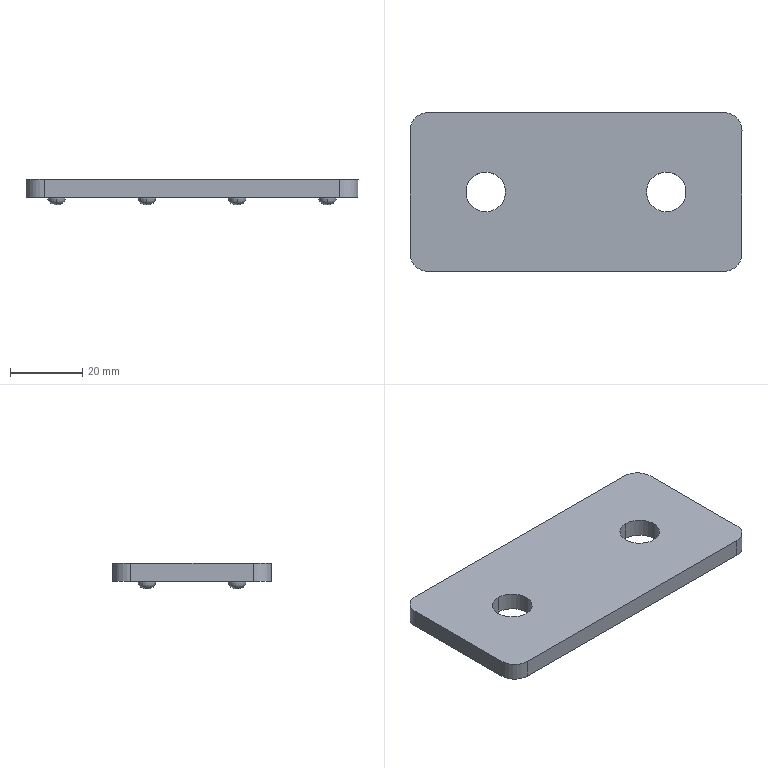Component | SolidWorks | G-Beam-1_BeamEndPlate-1 | 1 solid | 38 faces | box 92 x 44 x 7 mm | volume 19408 mm3 | torus 16 | plane 14 | cylinder 8 | commonest cylinder face diameters 11 x4 10 x4 | material Plain Carbon Steel
STEP:
#1=COLOUR_RGB('',0.7922,0.8196,0.9333);
#2=FILL_AREA_STYLE_COLOUR('',#1);
#3=FILL_AREA_STYLE('',(#2));
#4=SURFACE_STYLE_FILL_AREA(#3);
#5=SURFACE_SIDE_STYLE('',(#4));
#6=SURFACE_STYLE_USAGE(.BOTH.,#5);
#7=PRESENTATION_STYLE_ASSIGNMENT((#6));
#8=CARTESIAN_POINT('',(-170.63,344.077,264.226));
#9=VERTEX_POINT('',#8);
#10=CARTESIAN_POINT('',(-170.63,344.274,264.226));
#11=VERTEX_POINT('',#10);
#12=CARTESIAN_POINT('',(-170.63,344.176,264.226));
#13=DIRECTION('',(-0.,0.,-1.));
#14=DIRECTION('',(-0.,-1.,0.));
#15=AXIS2_PLACEMENT_3D('',#12,#13,#14);
#16=CIRCLE('',#15,0.09843);
#17=EDGE_CURVE('',#9,#11,#16,.T.);
#18=ORIENTED_EDGE('',*,*,#17,.T.);
#19=CARTESIAN_POINT('',(-170.63,344.195,264.147));
#20=VERTEX_POINT('',#19);
#21=CARTESIAN_POINT('',(-170.63,344.195,264.226));
#22=DIRECTION('',(-1.,0.,0.));
#23=DIRECTION('',(0.,0.,1.));
#24=AXIS2_PLACEMENT_3D('',#21,#22,#23);
#25=CIRCLE('',#24,0.07874);
#26=EDGE_CURVE('',#11,#20,#25,.T.);
#27=ORIENTED_EDGE('',*,*,#26,.T.);
#28=CARTESIAN_POINT('',(-170.63,344.156,264.147));
#29=VERTEX_POINT('',#28);
#30=CARTESIAN_POINT('',(-170.63,344.176,264.147));
#31=DIRECTION('',(-0.,0.,-1.));
#32=DIRECTION('',(-0.,-1.,0.));
#33=AXIS2_PLACEMENT_3D('',#30,#31,#32);
#34=CIRCLE('',#33,0.01969);
#35=EDGE_CURVE('',#29,#20,#34,.T.);
#36=ORIENTED_EDGE('',*,*,#35,.F.);
#37=CARTESIAN_POINT('',(-170.63,344.156,264.226));
#38=DIRECTION('',(1.,-0.,-0.));
#39=DIRECTION('',(-0.,0.,-1.));
#40=AXIS2_PLACEMENT_3D('',#37,#38,#39);
#41=CIRCLE('',#40,0.07874);
#42=EDGE_CURVE('',#9,#29,#41,.T.);
#43=ORIENTED_EDGE('',*,*,#42,.F.);
#44=EDGE_LOOP('',(#18,#27,#36,#43));
#45=FACE_OUTER_BOUND('',#44,.T.);
#46=CARTESIAN_POINT('',(-170.63,344.176,264.226));
#47=DIRECTION('',(-0.,0.,-1.));
#48=DIRECTION('',(-0.,-1.,-0.));
#49=AXIS2_PLACEMENT_3D('',#46,#47,#48);
#50=TOROIDAL_SURFACE('',#49,0.01969,0.07874);
#51=ADVANCED_FACE('',(#45),#50,.T.);
#52=CARTESIAN_POINT('',(-170.63,345.062,264.226));
#53=VERTEX_POINT('',#52);
#54=CARTESIAN_POINT('',(-170.63,345.258,264.226));
#55=VERTEX_POINT('',#54);
#56=CARTESIAN_POINT('',(-170.63,345.16,264.226));
#57=DIRECTION('',(-0.,0.,-1.));
#58=DIRECTION('',(-0.,-1.,0.));
#59=AXIS2_PLACEMENT_3D('',#56,#57,#58);
#60=CIRCLE('',#59,0.09843);
#61=EDGE_CURVE('',#53,#55,#60,.T.);
#62=ORIENTED_EDGE('',*,*,#61,.T.);
#63=CARTESIAN_POINT('',(-170.63,345.18,264.147));
#64=VERTEX_POINT('',#63);
#65=CARTESIAN_POINT('',(-170.63,345.18,264.226));
#66=DIRECTION('',(-1.,0.,0.));
#67=DIRECTION('',(0.,0.,1.));
#68=AXIS2_PLACEMENT_3D('',#65,#66,#67);
#69=CIRCLE('',#68,0.07874);
#70=EDGE_CURVE('',#55,#64,#69,.T.);
#71=ORIENTED_EDGE('',*,*,#70,.T.);
#72=CARTESIAN_POINT('',(-170.63,345.14,264.147));
#73=VERTEX_POINT('',#72);
#74=CARTESIAN_POINT('',(-170.63,345.16,264.147));
#75=DIRECTION('',(-0.,0.,-1.));
#76=DIRECTION('',(-0.,-1.,0.));
#77=AXIS2_PLACEMENT_3D('',#74,#75,#76);
#78=CIRCLE('',#77,0.01969);
#79=EDGE_CURVE('',#73,#64,#78,.T.);
#80=ORIENTED_EDGE('',*,*,#79,.F.);
#81=CARTESIAN_POINT('',(-170.63,345.14,264.226));
#82=DIRECTION('',(1.,-0.,-0.));
#83=DIRECTION('',(-0.,0.,-1.));
#84=AXIS2_PLACEMENT_3D('',#81,#82,#83);
#85=CIRCLE('',#84,0.07874);
#86=EDGE_CURVE('',#53,#73,#85,.T.);
#87=ORIENTED_EDGE('',*,*,#86,.F.);
#88=EDGE_LOOP('',(#62,#71,#80,#87));
#89=FACE_OUTER_BOUND('',#88,.T.);
#90=CARTESIAN_POINT('',(-170.63,345.16,264.226));
#91=DIRECTION('',(-0.,0.,-1.));
#92=DIRECTION('',(-0.,-1.,-0.));
#93=AXIS2_PLACEMENT_3D('',#90,#91,#92);
#94=TOROIDAL_SURFACE('',#93,0.01969,0.07874);
#95=ADVANCED_FACE('',(#89),#94,.T.);
#96=CARTESIAN_POINT('',(-171.614,344.077,264.226));
#97=VERTEX_POINT('',#96);
#98=CARTESIAN_POINT('',(-171.614,344.274,264.226));
#99=VERTEX_POINT('',#98);
#100=CARTESIAN_POINT('',(-171.614,344.176,264.226));
#101=DIRECTION('',(-0.,0.,-1.));
#102=DIRECTION('',(-0.,-1.,0.));
#103=AXIS2_PLACEMENT_3D('',#100,#101,#102);
#104=CIRCLE('',#103,0.09843);
#105=EDGE_CURVE('',#97,#99,#104,.T.);
#106=ORIENTED_EDGE('',*,*,#105,.T.);
#107=CARTESIAN_POINT('',(-171.614,344.195,264.147));
#108=VERTEX_POINT('',#107);
#109=CARTESIAN_POINT('',(-171.614,344.195,264.226));
#110=DIRECTION('',(-1.,0.,0.));
#111=DIRECTION('',(0.,0.,1.));
#112=AXIS2_PLACEMENT_3D('',#109,#110,#111);
#113=CIRCLE('',#112,0.07874);
#114=EDGE_CURVE('',#99,#108,#113,.T.);
#115=ORIENTED_EDGE('',*,*,#114,.T.);
#116=CARTESIAN_POINT('',(-171.614,344.156,264.147));
#117=VERTEX_POINT('',#116);
#118=CARTESIAN_POINT('',(-171.614,344.176,264.147));
#119=DIRECTION('',(-0.,0.,-1.));
#120=DIRECTION('',(-0.,-1.,0.));
#121=AXIS2_PLACEMENT_3D('',#118,#119,#120);
#122=CIRCLE('',#121,0.01969);
#123=EDGE_CURVE('',#117,#108,#122,.T.);
#124=ORIENTED_EDGE('',*,*,#123,.F.);
#125=CARTESIAN_POINT('',(-171.614,344.156,264.226));
#126=DIRECTION('',(1.,-0.,-0.));
#127=DIRECTION('',(-0.,0.,-1.));
#128=AXIS2_PLACEMENT_3D('',#125,#126,#127);
#129=CIRCLE('',#128,0.07874);
#130=EDGE_CURVE('',#97,#117,#129,.T.);
#131=ORIENTED_EDGE('',*,*,#130,.F.);
#132=EDGE_LOOP('',(#106,#115,#124,#131));
#133=FACE_OUTER_BOUND('',#132,.T.);
#134=CARTESIAN_POINT('',(-171.614,344.176,264.226));
#135=DIRECTION('',(-0.,0.,-1.));
#136=DIRECTION('',(-0.,-1.,-0.));
#137=AXIS2_PLACEMENT_3D('',#134,#135,#136);
#138=TOROIDAL_SURFACE('',#137,0.01969,0.07874);
#139=ADVANCED_FACE('',(#133),#138,.T.);
#140=CARTESIAN_POINT('',(-171.614,345.062,264.226));
#141=VERTEX_POINT('',#140);
#142=CARTESIAN_POINT('',(-171.614,345.258,264.226));
#143=VERTEX_POINT('',#142);
#144=CARTESIAN_POINT('',(-171.614,345.16,264.226));
#145=DIRECTION('',(-0.,0.,-1.));
#146=DIRECTION('',(-0.,-1.,0.));
#147=AXIS2_PLACEMENT_3D('',#144,#145,#146);
#148=CIRCLE('',#147,0.09843);
#149=EDGE_CURVE('',#141,#143,#148,.T.);
#150=ORIENTED_EDGE('',*,*,#149,.T.);
#151=CARTESIAN_POINT('',(-171.614,345.18,264.147));
#152=VERTEX_POINT('',#151);
#153=CARTESIAN_POINT('',(-171.614,345.18,264.226));
#154=DIRECTION('',(-1.,0.,0.));
#155=DIRECTION('',(0.,0.,1.));
#156=AXIS2_PLACEMENT_3D('',#153,#154,#155);
#157=CIRCLE('',#156,0.07874);
#158=EDGE_CURVE('',#143,#152,#157,.T.);
#159=ORIENTED_EDGE('',*,*,#158,.T.);
#160=CARTESIAN_POINT('',(-171.614,345.14,264.147));
#161=VERTEX_POINT('',#160);
#162=CARTESIAN_POINT('',(-171.614,345.16,264.147));
#163=DIRECTION('',(-0.,0.,-1.));
#164=DIRECTION('',(-0.,-1.,0.));
#165=AXIS2_PLACEMENT_3D('',#162,#163,#164);
#166=CIRCLE('',#165,0.01969);
#167=EDGE_CURVE('',#161,#152,#166,.T.);
#168=ORIENTED_EDGE('',*,*,#167,.F.);
#169=CARTESIAN_POINT('',(-171.614,345.14,264.226));
#170=DIRECTION('',(1.,-0.,-0.));
#171=DIRECTION('',(-0.,0.,-1.));
#172=AXIS2_PLACEMENT_3D('',#169,#170,#171);
#173=CIRCLE('',#172,0.07874);
#174=EDGE_CURVE('',#141,#161,#173,.T.);
#175=ORIENTED_EDGE('',*,*,#174,.F.);
#176=EDGE_LOOP('',(#150,#159,#168,#175));
#177=FACE_OUTER_BOUND('',#176,.T.);
#178=CARTESIAN_POINT('',(-171.614,345.16,264.226));
#179=DIRECTION('',(-0.,0.,-1.));
#180=DIRECTION('',(-0.,-1.,-0.));
#181=AXIS2_PLACEMENT_3D('',#178,#179,#180);
#182=TOROIDAL_SURFACE('',#181,0.01969,0.07874);
#183=ADVANCED_FACE('',(#177),#182,.T.);
#184=CARTESIAN_POINT('',(-172.599,344.156,264.147));
#185=VERTEX_POINT('',#184);
#186=CARTESIAN_POINT('',(-172.599,344.195,264.147));
#187=VERTEX_POINT('',#186);
#188=CARTESIAN_POINT('',(-172.599,344.176,264.147));
#189=DIRECTION('',(-0.,0.,-1.));
#190=DIRECTION('',(0.,1.,0.));
#191=AXIS2_PLACEMENT_3D('',#188,#189,#190);
#192=CIRCLE('',#191,0.01969);
#193=EDGE_CURVE('',#185,#187,#192,.T.);
#194=ORIENTED_EDGE('',*,*,#193,.F.);
#195=CARTESIAN_POINT('',(-172.599,344.077,264.226));
#196=VERTEX_POINT('',#195);
#197=CARTESIAN_POINT('',(-172.599,344.156,264.226));
#198=DIRECTION('',(-1.,0.,0.));
#199=DIRECTION('',(0.,0.,1.));
#200=AXIS2_PLACEMENT_3D('',#197,#198,#199);
#201=CIRCLE('',#200,0.07874);
#202=EDGE_CURVE('',#185,#196,#201,.T.);
#203=ORIENTED_EDGE('',*,*,#202,.T.);
#204=CARTESIAN_POINT('',(-172.599,344.274,264.226));
#205=VERTEX_POINT('',#204);
#206=CARTESIAN_POINT('',(-172.599,344.176,264.226));
#207=DIRECTION('',(-0.,0.,-1.));
#208=DIRECTION('',(-0.,-1.,0.));
#209=AXIS2_PLACEMENT_3D('',#206,#207,#208);
#210=CIRCLE('',#209,0.09843);
#211=EDGE_CURVE('',#196,#205,#210,.T.);
#212=ORIENTED_EDGE('',*,*,#211,.T.);
#213=CARTESIAN_POINT('',(-172.599,344.195,264.226));
#214=DIRECTION('',(1.,-0.,-0.));
#215=DIRECTION('',(-0.,0.,-1.));
#216=AXIS2_PLACEMENT_3D('',#213,#214,#215);
#217=CIRCLE('',#216,0.07874);
#218=EDGE_CURVE('',#187,#205,#217,.T.);
#219=ORIENTED_EDGE('',*,*,#218,.F.);
#220=EDGE_LOOP('',(#194,#203,#212,#219));
#221=FACE_OUTER_BOUND('',#220,.T.);
#222=CARTESIAN_POINT('',(-172.599,344.176,264.226));
#223=DIRECTION('',(0.,-0.,1.));
#224=DIRECTION('',(0.,1.,0.));
#225=AXIS2_PLACEMENT_3D('',#222,#223,#224);
#226=TOROIDAL_SURFACE('',#225,0.01969,0.07874);
#227=ADVANCED_FACE('',(#221),#226,.T.);
#228=CARTESIAN_POINT('',(-172.599,345.14,264.147));
#229=VERTEX_POINT('',#228);
#230=CARTESIAN_POINT('',(-172.599,345.18,264.147));
#231=VERTEX_POINT('',#230);
#232=CARTESIAN_POINT('',(-172.599,345.16,264.147));
#233=DIRECTION('',(-0.,0.,-1.));
#234=DIRECTION('',(0.,1.,0.));
#235=AXIS2_PLACEMENT_3D('',#232,#233,#234);
#236=CIRCLE('',#235,0.01969);
#237=EDGE_CURVE('',#229,#231,#236,.T.);
#238=ORIENTED_EDGE('',*,*,#237,.F.);
#239=CARTESIAN_POINT('',(-172.599,345.062,264.226));
#240=VERTEX_POINT('',#239);
#241=CARTESIAN_POINT('',(-172.599,345.14,264.226));
#242=DIRECTION('',(-1.,0.,0.));
#243=DIRECTION('',(0.,0.,1.));
#244=AXIS2_PLACEMENT_3D('',#241,#242,#243);
#245=CIRCLE('',#244,0.07874);
#246=EDGE_CURVE('',#229,#240,#245,.T.);
#247=ORIENTED_EDGE('',*,*,#246,.T.);
#248=CARTESIAN_POINT('',(-172.599,345.258,264.226));
#249=VERTEX_POINT('',#248);
#250=CARTESIAN_POINT('',(-172.599,345.16,264.226));
#251=DIRECTION('',(-0.,0.,-1.));
#252=DIRECTION('',(-0.,-1.,0.));
#253=AXIS2_PLACEMENT_3D('',#250,#251,#252);
#254=CIRCLE('',#253,0.09843);
#255=EDGE_CURVE('',#240,#249,#254,.T.);
#256=ORIENTED_EDGE('',*,*,#255,.T.);
#257=CARTESIAN_POINT('',(-172.599,345.18,264.226));
#258=DIRECTION('',(1.,-0.,-0.));
#259=DIRECTION('',(-0.,0.,-1.));
#260=AXIS2_PLACEMENT_3D('',#257,#258,#259);
#261=CIRCLE('',#260,0.07874);
#262=EDGE_CURVE('',#231,#249,#261,.T.);
#263=ORIENTED_EDGE('',*,*,#262,.F.);
#264=EDGE_LOOP('',(#238,#247,#256,#263));
#265=FACE_OUTER_BOUND('',#264,.T.);
#266=CARTESIAN_POINT('',(-172.599,345.16,264.226));
#267=DIRECTION('',(0.,-0.,1.));
#268=DIRECTION('',(0.,1.,0.));
#269=AXIS2_PLACEMENT_3D('',#266,#267,#268);
#270=TOROIDAL_SURFACE('',#269,0.01969,0.07874);
#271=ADVANCED_FACE('',(#265),#270,.T.);
#272=CARTESIAN_POINT('',(-173.583,344.156,264.147));
#273=VERTEX_POINT('',#272);
#274=CARTESIAN_POINT('',(-173.583,344.195,264.147));
#275=VERTEX_POINT('',#274);
#276=CARTESIAN_POINT('',(-173.583,344.176,264.147));
#277=DIRECTION('',(-0.,0.,-1.));
#278=DIRECTION('',(0.,1.,0.));
#279=AXIS2_PLACEMENT_3D('',#276,#277,#278);
#280=CIRCLE('',#279,0.01969);
#281=EDGE_CURVE('',#273,#275,#280,.T.);
#282=ORIENTED_EDGE('',*,*,#281,.F.);
#283=CARTESIAN_POINT('',(-173.583,344.077,264.226));
#284=VERTEX_POINT('',#283);
#285=CARTESIAN_POINT('',(-173.583,344.156,264.226));
#286=DIRECTION('',(-1.,0.,0.));
#287=DIRECTION('',(0.,0.,1.));
#288=AXIS2_PLACEMENT_3D('',#285,#286,#287);
#289=CIRCLE('',#288,0.07874);
#290=EDGE_CURVE('',#273,#284,#289,.T.);
#291=ORIENTED_EDGE('',*,*,#290,.T.);
#292=CARTESIAN_POINT('',(-173.583,344.274,264.226));
#293=VERTEX_POINT('',#292);
#294=CARTESIAN_POINT('',(-173.583,344.176,264.226));
#295=DIRECTION('',(-0.,0.,-1.));
#296=DIRECTION('',(-0.,-1.,0.));
#297=AXIS2_PLACEMENT_3D('',#294,#295,#296);
#298=CIRCLE('',#297,0.09843);
#299=EDGE_CURVE('',#284,#293,#298,.T.);
#300=ORIENTED_EDGE('',*,*,#299,.T.);
#301=CARTESIAN_POINT('',(-173.583,344.195,264.226));
#302=DIRECTION('',(1.,-0.,-0.));
#303=DIRECTION('',(-0.,0.,-1.));
#304=AXIS2_PLACEMENT_3D('',#301,#302,#303);
#305=CIRCLE('',#304,0.07874);
#306=EDGE_CURVE('',#275,#293,#305,.T.);
#307=ORIENTED_EDGE('',*,*,#306,.F.);
#308=EDGE_LOOP('',(#282,#291,#300,#307));
#309=FACE_OUTER_BOUND('',#308,.T.);
#310=CARTESIAN_POINT('',(-173.583,344.176,264.226));
#311=DIRECTION('',(0.,-0.,1.));
#312=DIRECTION('',(0.,1.,0.));
#313=AXIS2_PLACEMENT_3D('',#310,#311,#312);
#314=TOROIDAL_SURFACE('',#313,0.01969,0.07874);
#315=ADVANCED_FACE('',(#309),#314,.T.);
#316=CARTESIAN_POINT('',(-173.583,345.14,264.147));
#317=VERTEX_POINT('',#316);
#318=CARTESIAN_POINT('',(-173.583,345.18,264.147));
#319=VERTEX_POINT('',#318);
#320=CARTESIAN_POINT('',(-173.583,345.16,264.147));
#321=DIRECTION('',(-0.,0.,-1.));
#322=DIRECTION('',(0.,1.,0.));
#323=AXIS2_PLACEMENT_3D('',#320,#321,#322);
#324=CIRCLE('',#323,0.01969);
#325=EDGE_CURVE('',#317,#319,#324,.T.);
#326=ORIENTED_EDGE('',*,*,#325,.F.);
#327=CARTESIAN_POINT('',(-173.583,345.062,264.226));
#328=VERTEX_POINT('',#327);
#329=CARTESIAN_POINT('',(-173.583,345.14,264.226));
#330=DIRECTION('',(-1.,0.,0.));
#331=DIRECTION('',(0.,0.,1.));
#332=AXIS2_PLACEMENT_3D('',#329,#330,#331);
#333=CIRCLE('',#332,0.07874);
#334=EDGE_CURVE('',#317,#328,#333,.T.);
#335=ORIENTED_EDGE('',*,*,#334,.T.);
#336=CARTESIAN_POINT('',(-173.583,345.258,264.226));
#337=VERTEX_POINT('',#336);
#338=CARTESIAN_POINT('',(-173.583,345.16,264.226));
#339=DIRECTION('',(-0.,0.,-1.));
#340=DIRECTION('',(-0.,-1.,0.));
#341=AXIS2_PLACEMENT_3D('',#338,#339,#340);
#342=CIRCLE('',#341,0.09843);
#343=EDGE_CURVE('',#328,#337,#342,.T.);
#344=ORIENTED_EDGE('',*,*,#343,.T.);
#345=CARTESIAN_POINT('',(-173.583,345.18,264.226));
#346=DIRECTION('',(1.,-0.,-0.));
#347=DIRECTION('',(-0.,0.,-1.));
#348=AXIS2_PLACEMENT_3D('',#345,#346,#347);
#349=CIRCLE('',#348,0.07874);
#350=EDGE_CURVE('',#319,#337,#349,.T.);
#351=ORIENTED_EDGE('',*,*,#350,.F.);
#352=EDGE_LOOP('',(#326,#335,#344,#351));
#353=FACE_OUTER_BOUND('',#352,.T.);
#354=CARTESIAN_POINT('',(-173.583,345.16,264.226));
#355=DIRECTION('',(0.,-0.,1.));
#356=DIRECTION('',(0.,1.,0.));
#357=AXIS2_PLACEMENT_3D('',#354,#355,#356);
#358=TOROIDAL_SURFACE('',#357,0.01969,0.07874);
#359=ADVANCED_FACE('',(#353),#358,.T.);
#360=CARTESIAN_POINT('',(-173.091,344.884,264.226));
#361=VERTEX_POINT('',#360);
#362=CARTESIAN_POINT('',(-173.091,344.451,264.226));
#363=VERTEX_POINT('',#362);
#364=CARTESIAN_POINT('',(-173.091,344.668,264.226));
#365=DIRECTION('',(-0.,0.,-1.));
#366=DIRECTION('',(-0.,-1.,0.));
#367=AXIS2_PLACEMENT_3D('',#364,#365,#366);
#368=CIRCLE('',#367,0.2165);
#369=EDGE_CURVE('',#361,#363,#368,.T.);
#370=ORIENTED_EDGE('',*,*,#369,.T.);
#371=CARTESIAN_POINT('',(-173.091,344.451,264.423));
#372=VERTEX_POINT('',#371);
#373=CARTESIAN_POINT('',(-173.091,344.451,264.226));
#374=DIRECTION('',(0.,-0.,1.));
#375=VECTOR('',#374,39.37);
#376=LINE('',#373,#375);
#377=EDGE_CURVE('',#363,#372,#376,.T.);
#378=ORIENTED_EDGE('',*,*,#377,.T.);
#379=CARTESIAN_POINT('',(-173.091,344.884,264.423));
#380=VERTEX_POINT('',#379);
#381=CARTESIAN_POINT('',(-173.091,344.668,264.423));
#382=DIRECTION('',(-0.,0.,-1.));
#383=DIRECTION('',(-0.,-1.,0.));
#384=AXIS2_PLACEMENT_3D('',#381,#382,#383);
#385=CIRCLE('',#384,0.2165);
#386=EDGE_CURVE('',#380,#372,#385,.T.);
#387=ORIENTED_EDGE('',*,*,#386,.F.);
#388=CARTESIAN_POINT('',(-173.091,344.884,264.226));
#389=DIRECTION('',(0.,-0.,1.));
#390=VECTOR('',#389,39.37);
#391=LINE('',#388,#390);
#392=EDGE_CURVE('',#361,#380,#391,.T.);
#393=ORIENTED_EDGE('',*,*,#392,.F.);
#394=EDGE_LOOP('',(#370,#378,#387,#393));
#395=FACE_OUTER_BOUND('',#394,.T.);
#396=CARTESIAN_POINT('',(-173.091,344.668,264.226));
#397=DIRECTION('',(0.,-0.,1.));
#398=DIRECTION('',(0.,1.,0.));
#399=AXIS2_PLACEMENT_3D('',#396,#397,#398);
#400=CYLINDRICAL_SURFACE('',#399,0.2165);
#401=ADVANCED_FACE('',(#395),#400,.F.);
#402=CARTESIAN_POINT('',(-171.122,344.884,264.226));
#403=VERTEX_POINT('',#402);
#404=CARTESIAN_POINT('',(-171.122,344.451,264.226));
#405=VERTEX_POINT('',#404);
#406=CARTESIAN_POINT('',(-171.122,344.668,264.226));
#407=DIRECTION('',(-0.,0.,-1.));
#408=DIRECTION('',(-0.,-1.,0.));
#409=AXIS2_PLACEMENT_3D('',#406,#407,#408);
#410=CIRCLE('',#409,0.2165);
#411=EDGE_CURVE('',#403,#405,#410,.T.);
#412=ORIENTED_EDGE('',*,*,#411,.T.);
#413=CARTESIAN_POINT('',(-171.122,344.451,264.423));
#414=VERTEX_POINT('',#413);
#415=CARTESIAN_POINT('',(-171.122,344.451,264.226));
#416=DIRECTION('',(0.,-0.,1.));
#417=VECTOR('',#416,39.37);
#418=LINE('',#415,#417);
#419=EDGE_CURVE('',#405,#414,#418,.T.);
#420=ORIENTED_EDGE('',*,*,#419,.T.);
#421=CARTESIAN_POINT('',(-171.122,344.884,264.423));
#422=VERTEX_POINT('',#421);
#423=CARTESIAN_POINT('',(-171.122,344.668,264.423));
#424=DIRECTION('',(-0.,0.,-1.));
#425=DIRECTION('',(-0.,-1.,0.));
#426=AXIS2_PLACEMENT_3D('',#423,#424,#425);
#427=CIRCLE('',#426,0.2165);
#428=EDGE_CURVE('',#422,#414,#427,.T.);
#429=ORIENTED_EDGE('',*,*,#428,.F.);
#430=CARTESIAN_POINT('',(-171.122,344.884,264.226));
#431=DIRECTION('',(0.,-0.,1.));
#432=VECTOR('',#431,39.37);
#433=LINE('',#430,#432);
#434=EDGE_CURVE('',#403,#422,#433,.T.);
#435=ORIENTED_EDGE('',*,*,#434,.F.);
#436=EDGE_LOOP('',(#412,#420,#429,#435));
#437=FACE_OUTER_BOUND('',#436,.T.);
#438=CARTESIAN_POINT('',(-171.122,344.668,264.226));
#439=DIRECTION('',(0.,-0.,1.));
#440=DIRECTION('',(0.,1.,0.));
#441=AXIS2_PLACEMENT_3D('',#438,#439,#440);
#442=CYLINDRICAL_SURFACE('',#441,0.2165);
#443=ADVANCED_FACE('',(#437),#442,.F.);
#444=CARTESIAN_POINT('',(-172.599,345.16,264.226));
#445=DIRECTION('',(-0.,0.,-1.));
#446=DIRECTION('',(-0.,-1.,0.));
#447=AXIS2_PLACEMENT_3D('',#444,#445,#446);
#448=CIRCLE('',#447,0.09843);
#449=EDGE_CURVE('',#249,#240,#448,.T.);
#450=ORIENTED_EDGE('',*,*,#449,.F.);
#451=ORIENTED_EDGE('',*,*,#255,.F.);
#452=EDGE_LOOP('',(#450,#451));
#453=FACE_BOUND('',#452,.T.);
#454=ORIENTED_EDGE('',*,*,#17,.F.);
#455=CARTESIAN_POINT('',(-170.63,344.176,264.226));
#456=DIRECTION('',(-0.,0.,-1.));
#457=DIRECTION('',(-0.,-1.,0.));
#458=AXIS2_PLACEMENT_3D('',#455,#456,#457);
#459=CIRCLE('',#458,0.09843);
#460=EDGE_CURVE('',#11,#9,#459,.T.);
#461=ORIENTED_EDGE('',*,*,#460,.F.);
#462=EDGE_LOOP('',(#454,#461));
#463=FACE_BOUND('',#462,.T.);
#464=ORIENTED_EDGE('',*,*,#61,.F.);
#465=CARTESIAN_POINT('',(-170.63,345.16,264.226));
#466=DIRECTION('',(-0.,0.,-1.));
#467=DIRECTION('',(-0.,-1.,0.));
#468=AXIS2_PLACEMENT_3D('',#465,#466,#467);
#469=CIRCLE('',#468,0.09843);
#470=EDGE_CURVE('',#55,#53,#469,.T.);
#471=ORIENTED_EDGE('',*,*,#470,.F.);
#472=EDGE_LOOP('',(#464,#471));
#473=FACE_BOUND('',#472,.T.);
#474=ORIENTED_EDGE('',*,*,#105,.F.);
#475=CARTESIAN_POINT('',(-171.614,344.176,264.226));
#476=DIRECTION('',(-0.,0.,-1.));
#477=DIRECTION('',(-0.,-1.,0.));
#478=AXIS2_PLACEMENT_3D('',#475,#476,#477);
#479=CIRCLE('',#478,0.09843);
#480=EDGE_CURVE('',#99,#97,#479,.T.);
#481=ORIENTED_EDGE('',*,*,#480,.F.);
#482=EDGE_LOOP('',(#474,#481));
#483=FACE_BOUND('',#482,.T.);
#484=CARTESIAN_POINT('',(-172.599,344.176,264.226));
#485=DIRECTION('',(-0.,0.,-1.));
#486=DIRECTION('',(-0.,-1.,0.));
#487=AXIS2_PLACEMENT_3D('',#484,#485,#486);
#488=CIRCLE('',#487,0.09843);
#489=EDGE_CURVE('',#205,#196,#488,.T.);
#490=ORIENTED_EDGE('',*,*,#489,.F.);
#491=ORIENTED_EDGE('',*,*,#211,.F.);
#492=EDGE_LOOP('',(#490,#491));
#493=FACE_BOUND('',#492,.T.);
#494=CARTESIAN_POINT('',(-173.583,344.176,264.226));
#495=DIRECTION('',(-0.,0.,-1.));
#496=DIRECTION('',(-0.,-1.,0.));
#497=AXIS2_PLACEMENT_3D('',#494,#495,#496);
#498=CIRCLE('',#497,0.09843);
#499=EDGE_CURVE('',#293,#284,#498,.T.);
#500=ORIENTED_EDGE('',*,*,#499,.F.);
#501=ORIENTED_EDGE('',*,*,#299,.F.);
#502=EDGE_LOOP('',(#500,#501));
#503=FACE_BOUND('',#502,.T.);
#504=CARTESIAN_POINT('',(-173.583,345.16,264.226));
#505=DIRECTION('',(-0.,0.,-1.));
#506=DIRECTION('',(-0.,-1.,0.));
#507=AXIS2_PLACEMENT_3D('',#504,#505,#506);
#508=CIRCLE('',#507,0.09843);
#509=EDGE_CURVE('',#337,#328,#508,.T.);
#510=ORIENTED_EDGE('',*,*,#509,.F.);
#511=ORIENTED_EDGE('',*,*,#343,.F.);
#512=EDGE_LOOP('',(#510,#511));
#513=FACE_BOUND('',#512,.T.);
#514=ORIENTED_EDGE('',*,*,#149,.F.);
#515=CARTESIAN_POINT('',(-171.614,345.16,264.226));
#516=DIRECTION('',(-0.,0.,-1.));
#517=DIRECTION('',(-0.,-1.,0.));
#518=AXIS2_PLACEMENT_3D('',#515,#516,#517);
#519=CIRCLE('',#518,0.09843);
#520=EDGE_CURVE('',#143,#141,#519,.T.);
#521=ORIENTED_EDGE('',*,*,#520,.F.);
#522=EDGE_LOOP('',(#514,#521));
#523=FACE_BOUND('',#522,.T.);
#524=ORIENTED_EDGE('',*,*,#411,.F.);
#525=CARTESIAN_POINT('',(-171.122,344.668,264.226));
#526=DIRECTION('',(-0.,0.,-1.));
#527=DIRECTION('',(-0.,-1.,0.));
#528=AXIS2_PLACEMENT_3D('',#525,#526,#527);
#529=CIRCLE('',#528,0.2165);
#530=EDGE_CURVE('',#405,#403,#529,.T.);
#531=ORIENTED_EDGE('',*,*,#530,.F.);
#532=EDGE_LOOP('',(#524,#531));
#533=FACE_BOUND('',#532,.T.);
#534=CARTESIAN_POINT('',(-173.721,343.802,264.226));
#535=VERTEX_POINT('',#534);
#536=CARTESIAN_POINT('',(-173.917,343.999,264.226));
#537=VERTEX_POINT('',#536);
#538=CARTESIAN_POINT('',(-173.721,343.999,264.226));
#539=DIRECTION('',(-0.,0.,-1.));
#540=DIRECTION('',(-0.,-1.,0.));
#541=AXIS2_PLACEMENT_3D('',#538,#539,#540);
#542=CIRCLE('',#541,0.1969);
#543=EDGE_CURVE('',#535,#537,#542,.T.);
#544=ORIENTED_EDGE('',*,*,#543,.T.);
#545=CARTESIAN_POINT('',(-173.917,345.337,264.226));
#546=VERTEX_POINT('',#545);
#547=CARTESIAN_POINT('',(-173.917,345.337,264.226));
#548=DIRECTION('',(0.,1.,0.));
#549=VECTOR('',#548,39.37);
#550=LINE('',#547,#549);
#551=EDGE_CURVE('',#537,#546,#550,.T.);
#552=ORIENTED_EDGE('',*,*,#551,.T.);
#553=CARTESIAN_POINT('',(-173.721,345.534,264.226));
#554=VERTEX_POINT('',#553);
#555=CARTESIAN_POINT('',(-173.721,345.337,264.226));
#556=DIRECTION('',(-0.,0.,-1.));
#557=DIRECTION('',(-0.,-1.,0.));
#558=AXIS2_PLACEMENT_3D('',#555,#556,#557);
#559=CIRCLE('',#558,0.1969);
#560=EDGE_CURVE('',#546,#554,#559,.T.);
#561=ORIENTED_EDGE('',*,*,#560,.T.);
#562=CARTESIAN_POINT('',(-170.492,345.534,264.226));
#563=VERTEX_POINT('',#562);
#564=CARTESIAN_POINT('',(-170.492,345.534,264.226));
#565=DIRECTION('',(1.,-0.,-0.));
#566=VECTOR('',#565,39.37);
#567=LINE('',#564,#566);
#568=EDGE_CURVE('',#554,#563,#567,.T.);
#569=ORIENTED_EDGE('',*,*,#568,.T.);
#570=CARTESIAN_POINT('',(-170.295,345.337,264.226));
#571=VERTEX_POINT('',#570);
#572=CARTESIAN_POINT('',(-170.492,345.337,264.226));
#573=DIRECTION('',(-0.,0.,-1.));
#574=DIRECTION('',(0.,1.,0.));
#575=AXIS2_PLACEMENT_3D('',#572,#573,#574);
#576=CIRCLE('',#575,0.1969);
#577=EDGE_CURVE('',#563,#571,#576,.T.);
#578=ORIENTED_EDGE('',*,*,#577,.T.);
#579=CARTESIAN_POINT('',(-170.295,343.999,264.226));
#580=VERTEX_POINT('',#579);
#581=CARTESIAN_POINT('',(-170.295,345.337,264.226));
#582=DIRECTION('',(-0.,-1.,-0.));
#583=VECTOR('',#582,39.37);
#584=LINE('',#581,#583);
#585=EDGE_CURVE('',#571,#580,#584,.T.);
#586=ORIENTED_EDGE('',*,*,#585,.T.);
#587=CARTESIAN_POINT('',(-170.492,343.802,264.226));
#588=VERTEX_POINT('',#587);
#589=CARTESIAN_POINT('',(-170.492,343.999,264.226));
#590=DIRECTION('',(-0.,0.,-1.));
#591=DIRECTION('',(0.,1.,0.));
#592=AXIS2_PLACEMENT_3D('',#589,#590,#591);
#593=CIRCLE('',#592,0.1969);
#594=EDGE_CURVE('',#580,#588,#593,.T.);
#595=ORIENTED_EDGE('',*,*,#594,.T.);
#596=CARTESIAN_POINT('',(-170.492,343.802,264.226));
#597=DIRECTION('',(-1.,0.,0.));
#598=VECTOR('',#597,39.37);
#599=LINE('',#596,#598);
#600=EDGE_CURVE('',#588,#535,#599,.T.);
#601=ORIENTED_EDGE('',*,*,#600,.T.);
#602=EDGE_LOOP('',(#544,#552,#561,#569,#578,#586,#595,#601));
#603=FACE_OUTER_BOUND('',#602,.T.);
#604=ORIENTED_EDGE('',*,*,#369,.F.);
#605=CARTESIAN_POINT('',(-173.091,344.668,264.226));
#606=DIRECTION('',(-0.,0.,-1.));
#607=DIRECTION('',(-0.,-1.,0.));
#608=AXIS2_PLACEMENT_3D('',#605,#606,#607);
#609=CIRCLE('',#608,0.2165);
#610=EDGE_CURVE('',#363,#361,#609,.T.);
#611=ORIENTED_EDGE('',*,*,#610,.F.);
#612=EDGE_LOOP('',(#604,#611));
#613=FACE_BOUND('',#612,.T.);
#614=CARTESIAN_POINT('',(-173.721,343.999,264.226));
#615=DIRECTION('',(-0.,0.,-1.));
#616=DIRECTION('',(-0.,-1.,-0.));
#617=AXIS2_PLACEMENT_3D('',#614,#615,#616);
#618=PLANE('',#617);
#619=ADVANCED_FACE('',(#453,#463,#473,#483,#493,#503,#513,#523,#533,#603,#613),#618,.T.);
#620=ORIENTED_EDGE('',*,*,#428,.T.);
#621=CARTESIAN_POINT('',(-171.122,344.668,264.423));
#622=DIRECTION('',(-0.,0.,-1.));
#623=DIRECTION('',(-0.,-1.,0.));
#624=AXIS2_PLACEMENT_3D('',#621,#622,#623);
#625=CIRCLE('',#624,0.2165);
#626=EDGE_CURVE('',#414,#422,#625,.T.);
#627=ORIENTED_EDGE('',*,*,#626,.T.);
#628=EDGE_LOOP('',(#620,#627));
#629=FACE_BOUND('',#628,.T.);
#630=CARTESIAN_POINT('',(-173.721,343.802,264.423));
#631=VERTEX_POINT('',#630);
#632=CARTESIAN_POINT('',(-173.917,343.999,264.423));
#633=VERTEX_POINT('',#632);
#634=CARTESIAN_POINT('',(-173.721,343.999,264.423));
#635=DIRECTION('',(-0.,0.,-1.));
#636=DIRECTION('',(-0.,-1.,0.));
#637=AXIS2_PLACEMENT_3D('',#634,#635,#636);
#638=CIRCLE('',#637,0.1969);
#639=EDGE_CURVE('',#631,#633,#638,.T.);
#640=ORIENTED_EDGE('',*,*,#639,.F.);
#641=CARTESIAN_POINT('',(-170.492,343.802,264.423));
#642=VERTEX_POINT('',#641);
#643=CARTESIAN_POINT('',(-170.492,343.802,264.423));
#644=DIRECTION('',(-1.,0.,0.));
#645=VECTOR('',#644,39.37);
#646=LINE('',#643,#645);
#647=EDGE_CURVE('',#642,#631,#646,.T.);
#648=ORIENTED_EDGE('',*,*,#647,.F.);
#649=CARTESIAN_POINT('',(-170.295,343.999,264.423));
#650=VERTEX_POINT('',#649);
#651=CARTESIAN_POINT('',(-170.492,343.999,264.423));
#652=DIRECTION('',(-0.,0.,-1.));
#653=DIRECTION('',(0.,1.,0.));
#654=AXIS2_PLACEMENT_3D('',#651,#652,#653);
#655=CIRCLE('',#654,0.1969);
#656=EDGE_CURVE('',#650,#642,#655,.T.);
#657=ORIENTED_EDGE('',*,*,#656,.F.);
#658=CARTESIAN_POINT('',(-170.295,345.337,264.423));
#659=VERTEX_POINT('',#658);
#660=CARTESIAN_POINT('',(-170.295,345.337,264.423));
#661=DIRECTION('',(-0.,-1.,-0.));
#662=VECTOR('',#661,39.37);
#663=LINE('',#660,#662);
#664=EDGE_CURVE('',#659,#650,#663,.T.);
#665=ORIENTED_EDGE('',*,*,#664,.F.);
#666=CARTESIAN_POINT('',(-170.492,345.534,264.423));
#667=VERTEX_POINT('',#666);
#668=CARTESIAN_POINT('',(-170.492,345.337,264.423));
#669=DIRECTION('',(-0.,0.,-1.));
#670=DIRECTION('',(0.,1.,0.));
#671=AXIS2_PLACEMENT_3D('',#668,#669,#670);
#672=CIRCLE('',#671,0.1969);
#673=EDGE_CURVE('',#667,#659,#672,.T.);
#674=ORIENTED_EDGE('',*,*,#673,.F.);
#675=CARTESIAN_POINT('',(-173.721,345.534,264.423));
#676=VERTEX_POINT('',#675);
#677=CARTESIAN_POINT('',(-170.492,345.534,264.423));
#678=DIRECTION('',(1.,-0.,-0.));
#679=VECTOR('',#678,39.37);
#680=LINE('',#677,#679);
#681=EDGE_CURVE('',#676,#667,#680,.T.);
#682=ORIENTED_EDGE('',*,*,#681,.F.);
#683=CARTESIAN_POINT('',(-173.917,345.337,264.423));
#684=VERTEX_POINT('',#683);
#685=CARTESIAN_POINT('',(-173.721,345.337,264.423));
#686=DIRECTION('',(-0.,0.,-1.));
#687=DIRECTION('',(-0.,-1.,0.));
#688=AXIS2_PLACEMENT_3D('',#685,#686,#687);
#689=CIRCLE('',#688,0.1969);
#690=EDGE_CURVE('',#684,#676,#689,.T.);
#691=ORIENTED_EDGE('',*,*,#690,.F.);
#692=CARTESIAN_POINT('',(-173.917,345.337,264.423));
#693=DIRECTION('',(0.,1.,0.));
#694=VECTOR('',#693,39.37);
#695=LINE('',#692,#694);
#696=EDGE_CURVE('',#633,#684,#695,.T.);
#697=ORIENTED_EDGE('',*,*,#696,.F.);
#698=EDGE_LOOP('',(#640,#648,#657,#665,#674,#682,#691,#697));
#699=FACE_OUTER_BOUND('',#698,.T.);
#700=ORIENTED_EDGE('',*,*,#386,.T.);
#701=CARTESIAN_POINT('',(-173.091,344.668,264.423));
#702=DIRECTION('',(-0.,0.,-1.));
#703=DIRECTION('',(-0.,-1.,0.));
#704=AXIS2_PLACEMENT_3D('',#701,#702,#703);
#705=CIRCLE('',#704,0.2165);
#706=EDGE_CURVE('',#372,#380,#705,.T.);
#707=ORIENTED_EDGE('',*,*,#706,.T.);
#708=EDGE_LOOP('',(#700,#707));
#709=FACE_BOUND('',#708,.T.);
#710=CARTESIAN_POINT('',(-173.721,343.999,264.423));
#711=DIRECTION('',(-0.,0.,-1.));
#712=DIRECTION('',(-0.,-1.,-0.));
#713=AXIS2_PLACEMENT_3D('',#710,#711,#712);
#714=PLANE('',#713);
#715=ADVANCED_FACE('',(#629,#699,#709),#714,.F.);
#716=ORIENTED_EDGE('',*,*,#639,.T.);
#717=CARTESIAN_POINT('',(-173.917,343.999,264.226));
#718=DIRECTION('',(0.,-0.,1.));
#719=VECTOR('',#718,39.37);
#720=LINE('',#717,#719);
#721=EDGE_CURVE('',#537,#633,#720,.T.);
#722=ORIENTED_EDGE('',*,*,#721,.F.);
#723=ORIENTED_EDGE('',*,*,#543,.F.);
#724=CARTESIAN_POINT('',(-173.721,343.802,264.226));
#725=DIRECTION('',(0.,-0.,1.));
#726=VECTOR('',#725,39.37);
#727=LINE('',#724,#726);
#728=EDGE_CURVE('',#535,#631,#727,.T.);
#729=ORIENTED_EDGE('',*,*,#728,.T.);
#730=EDGE_LOOP('',(#716,#722,#723,#729));
#731=FACE_OUTER_BOUND('',#730,.T.);
#732=CARTESIAN_POINT('',(-173.721,343.999,264.226));
#733=DIRECTION('',(0.,-0.,1.));
#734=DIRECTION('',(0.,1.,0.));
#735=AXIS2_PLACEMENT_3D('',#732,#733,#734);
#736=CYLINDRICAL_SURFACE('',#735,0.1969);
#737=ADVANCED_FACE('',(#731),#736,.T.);
#738=ORIENTED_EDGE('',*,*,#696,.T.);
#739=CARTESIAN_POINT('',(-173.917,345.337,264.226));
#740=DIRECTION('',(0.,-0.,1.));
#741=VECTOR('',#740,39.37);
#742=LINE('',#739,#741);
#743=EDGE_CURVE('',#546,#684,#742,.T.);
#744=ORIENTED_EDGE('',*,*,#743,.F.);
#745=ORIENTED_EDGE('',*,*,#551,.F.);
#746=ORIENTED_EDGE('',*,*,#721,.T.);
#747=EDGE_LOOP('',(#738,#744,#745,#746));
#748=FACE_OUTER_BOUND('',#747,.T.);
#749=CARTESIAN_POINT('',(-173.917,345.337,264.226));
#750=DIRECTION('',(1.,-0.,-0.));
#751=DIRECTION('',(0.,-0.,1.));
#752=AXIS2_PLACEMENT_3D('',#749,#750,#751);
#753=PLANE('',#752);
#754=ADVANCED_FACE('',(#748),#753,.F.);
#755=ORIENTED_EDGE('',*,*,#690,.T.);
#756=CARTESIAN_POINT('',(-173.721,345.534,264.226));
#757=DIRECTION('',(0.,-0.,1.));
#758=VECTOR('',#757,39.37);
#759=LINE('',#756,#758);
#760=EDGE_CURVE('',#554,#676,#759,.T.);
#761=ORIENTED_EDGE('',*,*,#760,.F.);
#762=ORIENTED_EDGE('',*,*,#560,.F.);
#763=ORIENTED_EDGE('',*,*,#743,.T.);
#764=EDGE_LOOP('',(#755,#761,#762,#763));
#765=FACE_OUTER_BOUND('',#764,.T.);
#766=CARTESIAN_POINT('',(-173.721,345.337,264.226));
#767=DIRECTION('',(0.,-0.,1.));
#768=DIRECTION('',(0.,1.,0.));
#769=AXIS2_PLACEMENT_3D('',#766,#767,#768);
#770=CYLINDRICAL_SURFACE('',#769,0.1969);
#771=ADVANCED_FACE('',(#765),#770,.T.);
#772=ORIENTED_EDGE('',*,*,#681,.T.);
#773=CARTESIAN_POINT('',(-170.492,345.534,264.226));
#774=DIRECTION('',(0.,-0.,1.));
#775=VECTOR('',#774,39.37);
#776=LINE('',#773,#775);
#777=EDGE_CURVE('',#563,#667,#776,.T.);
#778=ORIENTED_EDGE('',*,*,#777,.F.);
#779=ORIENTED_EDGE('',*,*,#568,.F.);
#780=ORIENTED_EDGE('',*,*,#760,.T.);
#781=EDGE_LOOP('',(#772,#778,#779,#780));
#782=FACE_OUTER_BOUND('',#781,.T.);
#783=CARTESIAN_POINT('',(-170.492,345.534,264.226));
#784=DIRECTION('',(-0.,-1.,-0.));
#785=DIRECTION('',(0.,-0.,1.));
#786=AXIS2_PLACEMENT_3D('',#783,#784,#785);
#787=PLANE('',#786);
#788=ADVANCED_FACE('',(#782),#787,.F.);
#789=ORIENTED_EDGE('',*,*,#673,.T.);
#790=CARTESIAN_POINT('',(-170.295,345.337,264.226));
#791=DIRECTION('',(0.,-0.,1.));
#792=VECTOR('',#791,39.37);
#793=LINE('',#790,#792);
#794=EDGE_CURVE('',#571,#659,#793,.T.);
#795=ORIENTED_EDGE('',*,*,#794,.F.);
#796=ORIENTED_EDGE('',*,*,#577,.F.);
#797=ORIENTED_EDGE('',*,*,#777,.T.);
#798=EDGE_LOOP('',(#789,#795,#796,#797));
#799=FACE_OUTER_BOUND('',#798,.T.);
#800=CARTESIAN_POINT('',(-170.492,345.337,264.226));
#801=DIRECTION('',(0.,-0.,1.));
#802=DIRECTION('',(0.,1.,0.));
#803=AXIS2_PLACEMENT_3D('',#800,#801,#802);
#804=CYLINDRICAL_SURFACE('',#803,0.1969);
#805=ADVANCED_FACE('',(#799),#804,.T.);
#806=ORIENTED_EDGE('',*,*,#664,.T.);
#807=CARTESIAN_POINT('',(-170.295,343.999,264.226));
#808=DIRECTION('',(0.,-0.,1.));
#809=VECTOR('',#808,39.37);
#810=LINE('',#807,#809);
#811=EDGE_CURVE('',#580,#650,#810,.T.);
#812=ORIENTED_EDGE('',*,*,#811,.F.);
#813=ORIENTED_EDGE('',*,*,#585,.F.);
#814=ORIENTED_EDGE('',*,*,#794,.T.);
#815=EDGE_LOOP('',(#806,#812,#813,#814));
#816=FACE_OUTER_BOUND('',#815,.T.);
#817=CARTESIAN_POINT('',(-170.295,345.337,264.226));
#818=DIRECTION('',(-1.,0.,0.));
#819=DIRECTION('',(-0.,0.,-1.));
#820=AXIS2_PLACEMENT_3D('',#817,#818,#819);
#821=PLANE('',#820);
#822=ADVANCED_FACE('',(#816),#821,.F.);
#823=ORIENTED_EDGE('',*,*,#656,.T.);
#824=CARTESIAN_POINT('',(-170.492,343.802,264.226));
#825=DIRECTION('',(0.,-0.,1.));
#826=VECTOR('',#825,39.37);
#827=LINE('',#824,#826);
#828=EDGE_CURVE('',#588,#642,#827,.T.);
#829=ORIENTED_EDGE('',*,*,#828,.F.);
#830=ORIENTED_EDGE('',*,*,#594,.F.);
#831=ORIENTED_EDGE('',*,*,#811,.T.);
#832=EDGE_LOOP('',(#823,#829,#830,#831));
#833=FACE_OUTER_BOUND('',#832,.T.);
#834=CARTESIAN_POINT('',(-170.492,343.999,264.226));
#835=DIRECTION('',(0.,-0.,1.));
#836=DIRECTION('',(0.,1.,0.));
#837=AXIS2_PLACEMENT_3D('',#834,#835,#836);
#838=CYLINDRICAL_SURFACE('',#837,0.1969);
#839=ADVANCED_FACE('',(#833),#838,.T.);
#840=ORIENTED_EDGE('',*,*,#647,.T.);
#841=ORIENTED_EDGE('',*,*,#728,.F.);
#842=ORIENTED_EDGE('',*,*,#600,.F.);
#843=ORIENTED_EDGE('',*,*,#828,.T.);
#844=EDGE_LOOP('',(#840,#841,#842,#843));
#845=FACE_OUTER_BOUND('',#844,.T.);
#846=CARTESIAN_POINT('',(-170.492,343.802,264.226));
#847=DIRECTION('',(0.,1.,0.));
#848=DIRECTION('',(-0.,0.,-1.));
#849=AXIS2_PLACEMENT_3D('',#846,#847,#848);
#850=PLANE('',#849);
#851=ADVANCED_FACE('',(#845),#850,.F.);
#852=ORIENTED_EDGE('',*,*,#419,.F.);
#853=ORIENTED_EDGE('',*,*,#530,.T.);
#854=ORIENTED_EDGE('',*,*,#434,.T.);
#855=ORIENTED_EDGE('',*,*,#626,.F.);
#856=EDGE_LOOP('',(#852,#853,#854,#855));
#857=FACE_OUTER_BOUND('',#856,.T.);
#858=CARTESIAN_POINT('',(-171.122,344.668,264.226));
#859=DIRECTION('',(0.,-0.,1.));
#860=DIRECTION('',(0.,1.,0.));
#861=AXIS2_PLACEMENT_3D('',#858,#859,#860);
#862=CYLINDRICAL_SURFACE('',#861,0.2165);
#863=ADVANCED_FACE('',(#857),#862,.F.);
#864=ORIENTED_EDGE('',*,*,#377,.F.);
#865=ORIENTED_EDGE('',*,*,#610,.T.);
#866=ORIENTED_EDGE('',*,*,#392,.T.);
#867=ORIENTED_EDGE('',*,*,#706,.F.);
#868=EDGE_LOOP('',(#864,#865,#866,#867));
#869=FACE_OUTER_BOUND('',#868,.T.);
#870=CARTESIAN_POINT('',(-173.091,344.668,264.226));
#871=DIRECTION('',(0.,-0.,1.));
#872=DIRECTION('',(0.,1.,0.));
#873=AXIS2_PLACEMENT_3D('',#870,#871,#872);
#874=CYLINDRICAL_SURFACE('',#873,0.2165);
#875=ADVANCED_FACE('',(#869),#874,.F.);
#876=ORIENTED_EDGE('',*,*,#167,.T.);
#877=CARTESIAN_POINT('',(-171.614,345.16,264.147));
#878=DIRECTION('',(-0.,0.,-1.));
#879=DIRECTION('',(-0.,-1.,0.));
#880=AXIS2_PLACEMENT_3D('',#877,#878,#879);
#881=CIRCLE('',#880,0.01969);
#882=EDGE_CURVE('',#152,#161,#881,.T.);
#883=ORIENTED_EDGE('',*,*,#882,.T.);
#884=EDGE_LOOP('',(#876,#883));
#885=FACE_OUTER_BOUND('',#884,.T.);
#886=CARTESIAN_POINT('',(-171.614,345.16,264.147));
#887=DIRECTION('',(-0.,0.,-1.));
#888=DIRECTION('',(-0.,-1.,-0.));
#889=AXIS2_PLACEMENT_3D('',#886,#887,#888);
#890=PLANE('',#889);
#891=ADVANCED_FACE('',(#885),#890,.T.);
#892=CARTESIAN_POINT('',(-173.583,345.16,264.147));
#893=DIRECTION('',(-0.,0.,-1.));
#894=DIRECTION('',(0.,1.,0.));
#895=AXIS2_PLACEMENT_3D('',#892,#893,#894);
#896=CIRCLE('',#895,0.01969);
#897=EDGE_CURVE('',#319,#317,#896,.T.);
#898=ORIENTED_EDGE('',*,*,#897,.T.);
#899=ORIENTED_EDGE('',*,*,#325,.T.);
#900=EDGE_LOOP('',(#898,#899));
#901=FACE_OUTER_BOUND('',#900,.T.);
#902=CARTESIAN_POINT('',(-173.583,345.16,264.147));
#903=DIRECTION('',(0.,-0.,1.));
#904=DIRECTION('',(0.,1.,0.));
#905=AXIS2_PLACEMENT_3D('',#902,#903,#904);
#906=PLANE('',#905);
#907=ADVANCED_FACE('',(#901),#906,.F.);
#908=CARTESIAN_POINT('',(-173.583,344.176,264.147));
#909=DIRECTION('',(-0.,0.,-1.));
#910=DIRECTION('',(0.,1.,0.));
#911=AXIS2_PLACEMENT_3D('',#908,#909,#910);
#912=CIRCLE('',#911,0.01969);
#913=EDGE_CURVE('',#275,#273,#912,.T.);
#914=ORIENTED_EDGE('',*,*,#913,.T.);
#915=ORIENTED_EDGE('',*,*,#281,.T.);
#916=EDGE_LOOP('',(#914,#915));
#917=FACE_OUTER_BOUND('',#916,.T.);
#918=CARTESIAN_POINT('',(-173.583,344.176,264.147));
#919=DIRECTION('',(0.,-0.,1.));
#920=DIRECTION('',(0.,1.,0.));
#921=AXIS2_PLACEMENT_3D('',#918,#919,#920);
#922=PLANE('',#921);
#923=ADVANCED_FACE('',(#917),#922,.F.);
#924=CARTESIAN_POINT('',(-172.599,344.176,264.147));
#925=DIRECTION('',(-0.,0.,-1.));
#926=DIRECTION('',(0.,1.,0.));
#927=AXIS2_PLACEMENT_3D('',#924,#925,#926);
#928=CIRCLE('',#927,0.01969);
#929=EDGE_CURVE('',#187,#185,#928,.T.);
#930=ORIENTED_EDGE('',*,*,#929,.T.);
#931=ORIENTED_EDGE('',*,*,#193,.T.);
#932=EDGE_LOOP('',(#930,#931));
#933=FACE_OUTER_BOUND('',#932,.T.);
#934=CARTESIAN_POINT('',(-172.599,344.176,264.147));
#935=DIRECTION('',(0.,-0.,1.));
#936=DIRECTION('',(0.,1.,0.));
#937=AXIS2_PLACEMENT_3D('',#934,#935,#936);
#938=PLANE('',#937);
#939=ADVANCED_FACE('',(#933),#938,.F.);
#940=ORIENTED_EDGE('',*,*,#123,.T.);
#941=CARTESIAN_POINT('',(-171.614,344.176,264.147));
#942=DIRECTION('',(-0.,0.,-1.));
#943=DIRECTION('',(-0.,-1.,0.));
#944=AXIS2_PLACEMENT_3D('',#941,#942,#943);
#945=CIRCLE('',#944,0.01969);
#946=EDGE_CURVE('',#108,#117,#945,.T.);
#947=ORIENTED_EDGE('',*,*,#946,.T.);
#948=EDGE_LOOP('',(#940,#947));
#949=FACE_OUTER_BOUND('',#948,.T.);
#950=CARTESIAN_POINT('',(-171.614,344.176,264.147));
#951=DIRECTION('',(-0.,0.,-1.));
#952=DIRECTION('',(-0.,-1.,-0.));
#953=AXIS2_PLACEMENT_3D('',#950,#951,#952);
#954=PLANE('',#953);
#955=ADVANCED_FACE('',(#949),#954,.T.);
#956=ORIENTED_EDGE('',*,*,#79,.T.);
#957=CARTESIAN_POINT('',(-170.63,345.16,264.147));
#958=DIRECTION('',(-0.,0.,-1.));
#959=DIRECTION('',(-0.,-1.,0.));
#960=AXIS2_PLACEMENT_3D('',#957,#958,#959);
#961=CIRCLE('',#960,0.01969);
#962=EDGE_CURVE('',#64,#73,#961,.T.);
#963=ORIENTED_EDGE('',*,*,#962,.T.);
#964=EDGE_LOOP('',(#956,#963));
#965=FACE_OUTER_BOUND('',#964,.T.);
#966=CARTESIAN_POINT('',(-170.63,345.16,264.147));
#967=DIRECTION('',(-0.,0.,-1.));
#968=DIRECTION('',(-0.,-1.,-0.));
#969=AXIS2_PLACEMENT_3D('',#966,#967,#968);
#970=PLANE('',#969);
#971=ADVANCED_FACE('',(#965),#970,.T.);
#972=ORIENTED_EDGE('',*,*,#35,.T.);
#973=CARTESIAN_POINT('',(-170.63,344.176,264.147));
#974=DIRECTION('',(-0.,0.,-1.));
#975=DIRECTION('',(-0.,-1.,0.));
#976=AXIS2_PLACEMENT_3D('',#973,#974,#975);
#977=CIRCLE('',#976,0.01969);
#978=EDGE_CURVE('',#20,#29,#977,.T.);
#979=ORIENTED_EDGE('',*,*,#978,.T.);
#980=EDGE_LOOP('',(#972,#979));
#981=FACE_OUTER_BOUND('',#980,.T.);
#982=CARTESIAN_POINT('',(-170.63,344.176,264.147));
#983=DIRECTION('',(-0.,0.,-1.));
#984=DIRECTION('',(-0.,-1.,-0.));
#985=AXIS2_PLACEMENT_3D('',#982,#983,#984);
#986=PLANE('',#985);
#987=ADVANCED_FACE('',(#981),#986,.T.);
#988=CARTESIAN_POINT('',(-172.599,345.16,264.147));
#989=DIRECTION('',(-0.,0.,-1.));
#990=DIRECTION('',(0.,1.,0.));
#991=AXIS2_PLACEMENT_3D('',#988,#989,#990);
#992=CIRCLE('',#991,0.01969);
#993=EDGE_CURVE('',#231,#229,#992,.T.);
#994=ORIENTED_EDGE('',*,*,#993,.T.);
#995=ORIENTED_EDGE('',*,*,#237,.T.);
#996=EDGE_LOOP('',(#994,#995));
#997=FACE_OUTER_BOUND('',#996,.T.);
#998=CARTESIAN_POINT('',(-172.599,345.16,264.147));
#999=DIRECTION('',(0.,-0.,1.));
#1000=DIRECTION('',(0.,1.,0.));
#1001=AXIS2_PLACEMENT_3D('',#998,#999,#1000);
#1002=PLANE('',#1001);
#1003=ADVANCED_FACE('',(#997),#1002,.F.);
#1004=ORIENTED_EDGE('',*,*,#334,.F.);
#1005=ORIENTED_EDGE('',*,*,#897,.F.);
#1006=ORIENTED_EDGE('',*,*,#350,.T.);
#1007=ORIENTED_EDGE('',*,*,#509,.T.);
#1008=EDGE_LOOP('',(#1004,#1005,#1006,#1007));
#1009=FACE_OUTER_BOUND('',#1008,.T.);
#1010=CARTESIAN_POINT('',(-173.583,345.16,264.226));
#1011=DIRECTION('',(0.,-0.,1.));
#1012=DIRECTION('',(0.,1.,0.));
#1013=AXIS2_PLACEMENT_3D('',#1010,#1011,#1012);
#1014=TOROIDAL_SURFACE('',#1013,0.01969,0.07874);
#1015=ADVANCED_FACE('',(#1009),#1014,.T.);
#1016=ORIENTED_EDGE('',*,*,#290,.F.);
#1017=ORIENTED_EDGE('',*,*,#913,.F.);
#1018=ORIENTED_EDGE('',*,*,#306,.T.);
#1019=ORIENTED_EDGE('',*,*,#499,.T.);
#1020=EDGE_LOOP('',(#1016,#1017,#1018,#1019));
#1021=FACE_OUTER_BOUND('',#1020,.T.);
#1022=CARTESIAN_POINT('',(-173.583,344.176,264.226));
#1023=DIRECTION('',(0.,-0.,1.));
#1024=DIRECTION('',(0.,1.,0.));
#1025=AXIS2_PLACEMENT_3D('',#1022,#1023,#1024);
#1026=TOROIDAL_SURFACE('',#1025,0.01969,0.07874);
#1027=ADVANCED_FACE('',(#1021),#1026,.T.);
#1028=ORIENTED_EDGE('',*,*,#246,.F.);
#1029=ORIENTED_EDGE('',*,*,#993,.F.);
#1030=ORIENTED_EDGE('',*,*,#262,.T.);
#1031=ORIENTED_EDGE('',*,*,#449,.T.);
#1032=EDGE_LOOP('',(#1028,#1029,#1030,#1031));
#1033=FACE_OUTER_BOUND('',#1032,.T.);
#1034=CARTESIAN_POINT('',(-172.599,345.16,264.226));
#1035=DIRECTION('',(0.,-0.,1.));
#1036=DIRECTION('',(0.,1.,0.));
#1037=AXIS2_PLACEMENT_3D('',#1034,#1035,#1036);
#1038=TOROIDAL_SURFACE('',#1037,0.01969,0.07874);
#1039=ADVANCED_FACE('',(#1033),#1038,.T.);
#1040=ORIENTED_EDGE('',*,*,#202,.F.);
#1041=ORIENTED_EDGE('',*,*,#929,.F.);
#1042=ORIENTED_EDGE('',*,*,#218,.T.);
#1043=ORIENTED_EDGE('',*,*,#489,.T.);
#1044=EDGE_LOOP('',(#1040,#1041,#1042,#1043));
#1045=FACE_OUTER_BOUND('',#1044,.T.);
#1046=CARTESIAN_POINT('',(-172.599,344.176,264.226));
#1047=DIRECTION('',(0.,-0.,1.));
#1048=DIRECTION('',(0.,1.,0.));
#1049=AXIS2_PLACEMENT_3D('',#1046,#1047,#1048);
#1050=TOROIDAL_SURFACE('',#1049,0.01969,0.07874);
#1051=ADVANCED_FACE('',(#1045),#1050,.T.);
#1052=ORIENTED_EDGE('',*,*,#158,.F.);
#1053=ORIENTED_EDGE('',*,*,#520,.T.);
#1054=ORIENTED_EDGE('',*,*,#174,.T.);
#1055=ORIENTED_EDGE('',*,*,#882,.F.);
#1056=EDGE_LOOP('',(#1052,#1053,#1054,#1055));
#1057=FACE_OUTER_BOUND('',#1056,.T.);
#1058=CARTESIAN_POINT('',(-171.614,345.16,264.226));
#1059=DIRECTION('',(-0.,0.,-1.));
#1060=DIRECTION('',(-0.,-1.,-0.));
#1061=AXIS2_PLACEMENT_3D('',#1058,#1059,#1060);
#1062=TOROIDAL_SURFACE('',#1061,0.01969,0.07874);
#1063=ADVANCED_FACE('',(#1057),#1062,.T.);
#1064=ORIENTED_EDGE('',*,*,#114,.F.);
#1065=ORIENTED_EDGE('',*,*,#480,.T.);
#1066=ORIENTED_EDGE('',*,*,#130,.T.);
#1067=ORIENTED_EDGE('',*,*,#946,.F.);
#1068=EDGE_LOOP('',(#1064,#1065,#1066,#1067));
#1069=FACE_OUTER_BOUND('',#1068,.T.);
#1070=CARTESIAN_POINT('',(-171.614,344.176,264.226));
#1071=DIRECTION('',(-0.,0.,-1.));
#1072=DIRECTION('',(-0.,-1.,-0.));
#1073=AXIS2_PLACEMENT_3D('',#1070,#1071,#1072);
#1074=TOROIDAL_SURFACE('',#1073,0.01969,0.07874);
#1075=ADVANCED_FACE('',(#1069),#1074,.T.);
#1076=ORIENTED_EDGE('',*,*,#70,.F.);
#1077=ORIENTED_EDGE('',*,*,#470,.T.);
#1078=ORIENTED_EDGE('',*,*,#86,.T.);
#1079=ORIENTED_EDGE('',*,*,#962,.F.);
#1080=EDGE_LOOP('',(#1076,#1077,#1078,#1079));
#1081=FACE_OUTER_BOUND('',#1080,.T.);
#1082=CARTESIAN_POINT('',(-170.63,345.16,264.226));
#1083=DIRECTION('',(-0.,0.,-1.));
#1084=DIRECTION('',(-0.,-1.,-0.));
#1085=AXIS2_PLACEMENT_3D('',#1082,#1083,#1084);
#1086=TOROIDAL_SURFACE('',#1085,0.01969,0.07874);
#1087=ADVANCED_FACE('',(#1081),#1086,.T.);
#1088=ORIENTED_EDGE('',*,*,#26,.F.);
#1089=ORIENTED_EDGE('',*,*,#460,.T.);
#1090=ORIENTED_EDGE('',*,*,#42,.T.);
#1091=ORIENTED_EDGE('',*,*,#978,.F.);
#1092=EDGE_LOOP('',(#1088,#1089,#1090,#1091));
#1093=FACE_OUTER_BOUND('',#1092,.T.);
#1094=CARTESIAN_POINT('',(-170.63,344.176,264.226));
#1095=DIRECTION('',(-0.,0.,-1.));
#1096=DIRECTION('',(-0.,-1.,-0.));
#1097=AXIS2_PLACEMENT_3D('',#1094,#1095,#1096);
#1098=TOROIDAL_SURFACE('',#1097,0.01969,0.07874);
#1099=ADVANCED_FACE('',(#1093),#1098,.T.);
#1100=CLOSED_SHELL('',(#51,#95,#139,#183,#227,#271,#315,#359,#401,#443,#619,#715,#737,#754,#771,#788,#805,#822,#839,#851,#863,#875,#891,#907,#923,#939,#955,#971,#987,#1003,#1015,#1027,#1039,#1051,#1063,#1075,#1087,#1099));
#1101=MANIFOLD_SOLID_BREP('',#1100);
#1102=STYLED_ITEM('',(#7),#1101);
#1103=PRESENTATION_LAYER_ASSIGNMENT('','',(#1102));
#1104=(LENGTH_UNIT()NAMED_UNIT(*)SI_UNIT($,.METRE.));
#1105=LENGTH_MEASURE_WITH_UNIT(LENGTH_MEASURE(0.0254),#1104);
#1106=DIMENSIONAL_EXPONENTS(1.,0.,0.,0.,0.,0.,0.);
#1107=(CONVERSION_BASED_UNIT('',#1105)LENGTH_UNIT()NAMED_UNIT(#1106));
#1108=UNCERTAINTY_MEASURE_WITH_UNIT(LENGTH_MEASURE(0.00001),#1107,'','');
#1109=(NAMED_UNIT(*)PLANE_ANGLE_UNIT()SI_UNIT($,.RADIAN.));
#1110=(NAMED_UNIT(*)SI_UNIT($,.STERADIAN.)SOLID_ANGLE_UNIT());
#1111=(GEOMETRIC_REPRESENTATION_CONTEXT(3)GLOBAL_UNCERTAINTY_ASSIGNED_CONTEXT((#1108))GLOBAL_UNIT_ASSIGNED_CONTEXT((#1107,#1109,#1110))REPRESENTATION_CONTEXT('',''));
#1112=MECHANICAL_DESIGN_GEOMETRIC_PRESENTATION_REPRESENTATION('',(#1102),#1111);
#1113=CARTESIAN_POINT('',(0.,0.,0.));
#1114=DIRECTION('',(0.,0.,1.));
#1115=DIRECTION('',(1.,0.,0.));
#1116=AXIS2_PLACEMENT_3D('',#1113,#1114,#1115);
#1117=(LENGTH_UNIT()NAMED_UNIT(*)SI_UNIT($,.METRE.));
#1118=LENGTH_MEASURE_WITH_UNIT(LENGTH_MEASURE(0.0254),#1117);
#1119=DIMENSIONAL_EXPONENTS(1.,0.,0.,0.,0.,0.,0.);
#1120=(CONVERSION_BASED_UNIT('',#1118)LENGTH_UNIT()NAMED_UNIT(#1119));
#1121=UNCERTAINTY_MEASURE_WITH_UNIT(LENGTH_MEASURE(0.00001),#1120,'','');
#1122=(NAMED_UNIT(*)PLANE_ANGLE_UNIT()SI_UNIT($,.RADIAN.));
#1123=(NAMED_UNIT(*)SI_UNIT($,.STERADIAN.)SOLID_ANGLE_UNIT());
#1124=(GEOMETRIC_REPRESENTATION_CONTEXT(3)GLOBAL_UNCERTAINTY_ASSIGNED_CONTEXT((#1121))GLOBAL_UNIT_ASSIGNED_CONTEXT((#1120,#1122,#1123))REPRESENTATION_CONTEXT('',''));
#1125=ADVANCED_BREP_SHAPE_REPRESENTATION('',(#1101,#1116),#1124);